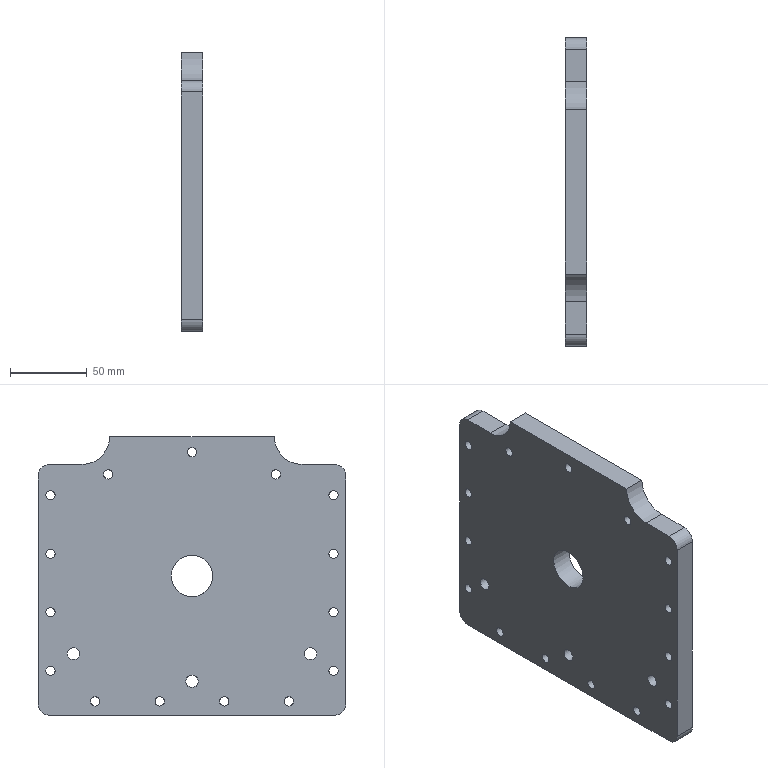Component | NX | FRONT_END_CAP | 1 solid | 33 faces | volume 468570 mm3 | cylinder 25 | plane 8 | commonest cylinder face diameters 6 x15 15 x4 8 x3 36 x2 27 x1